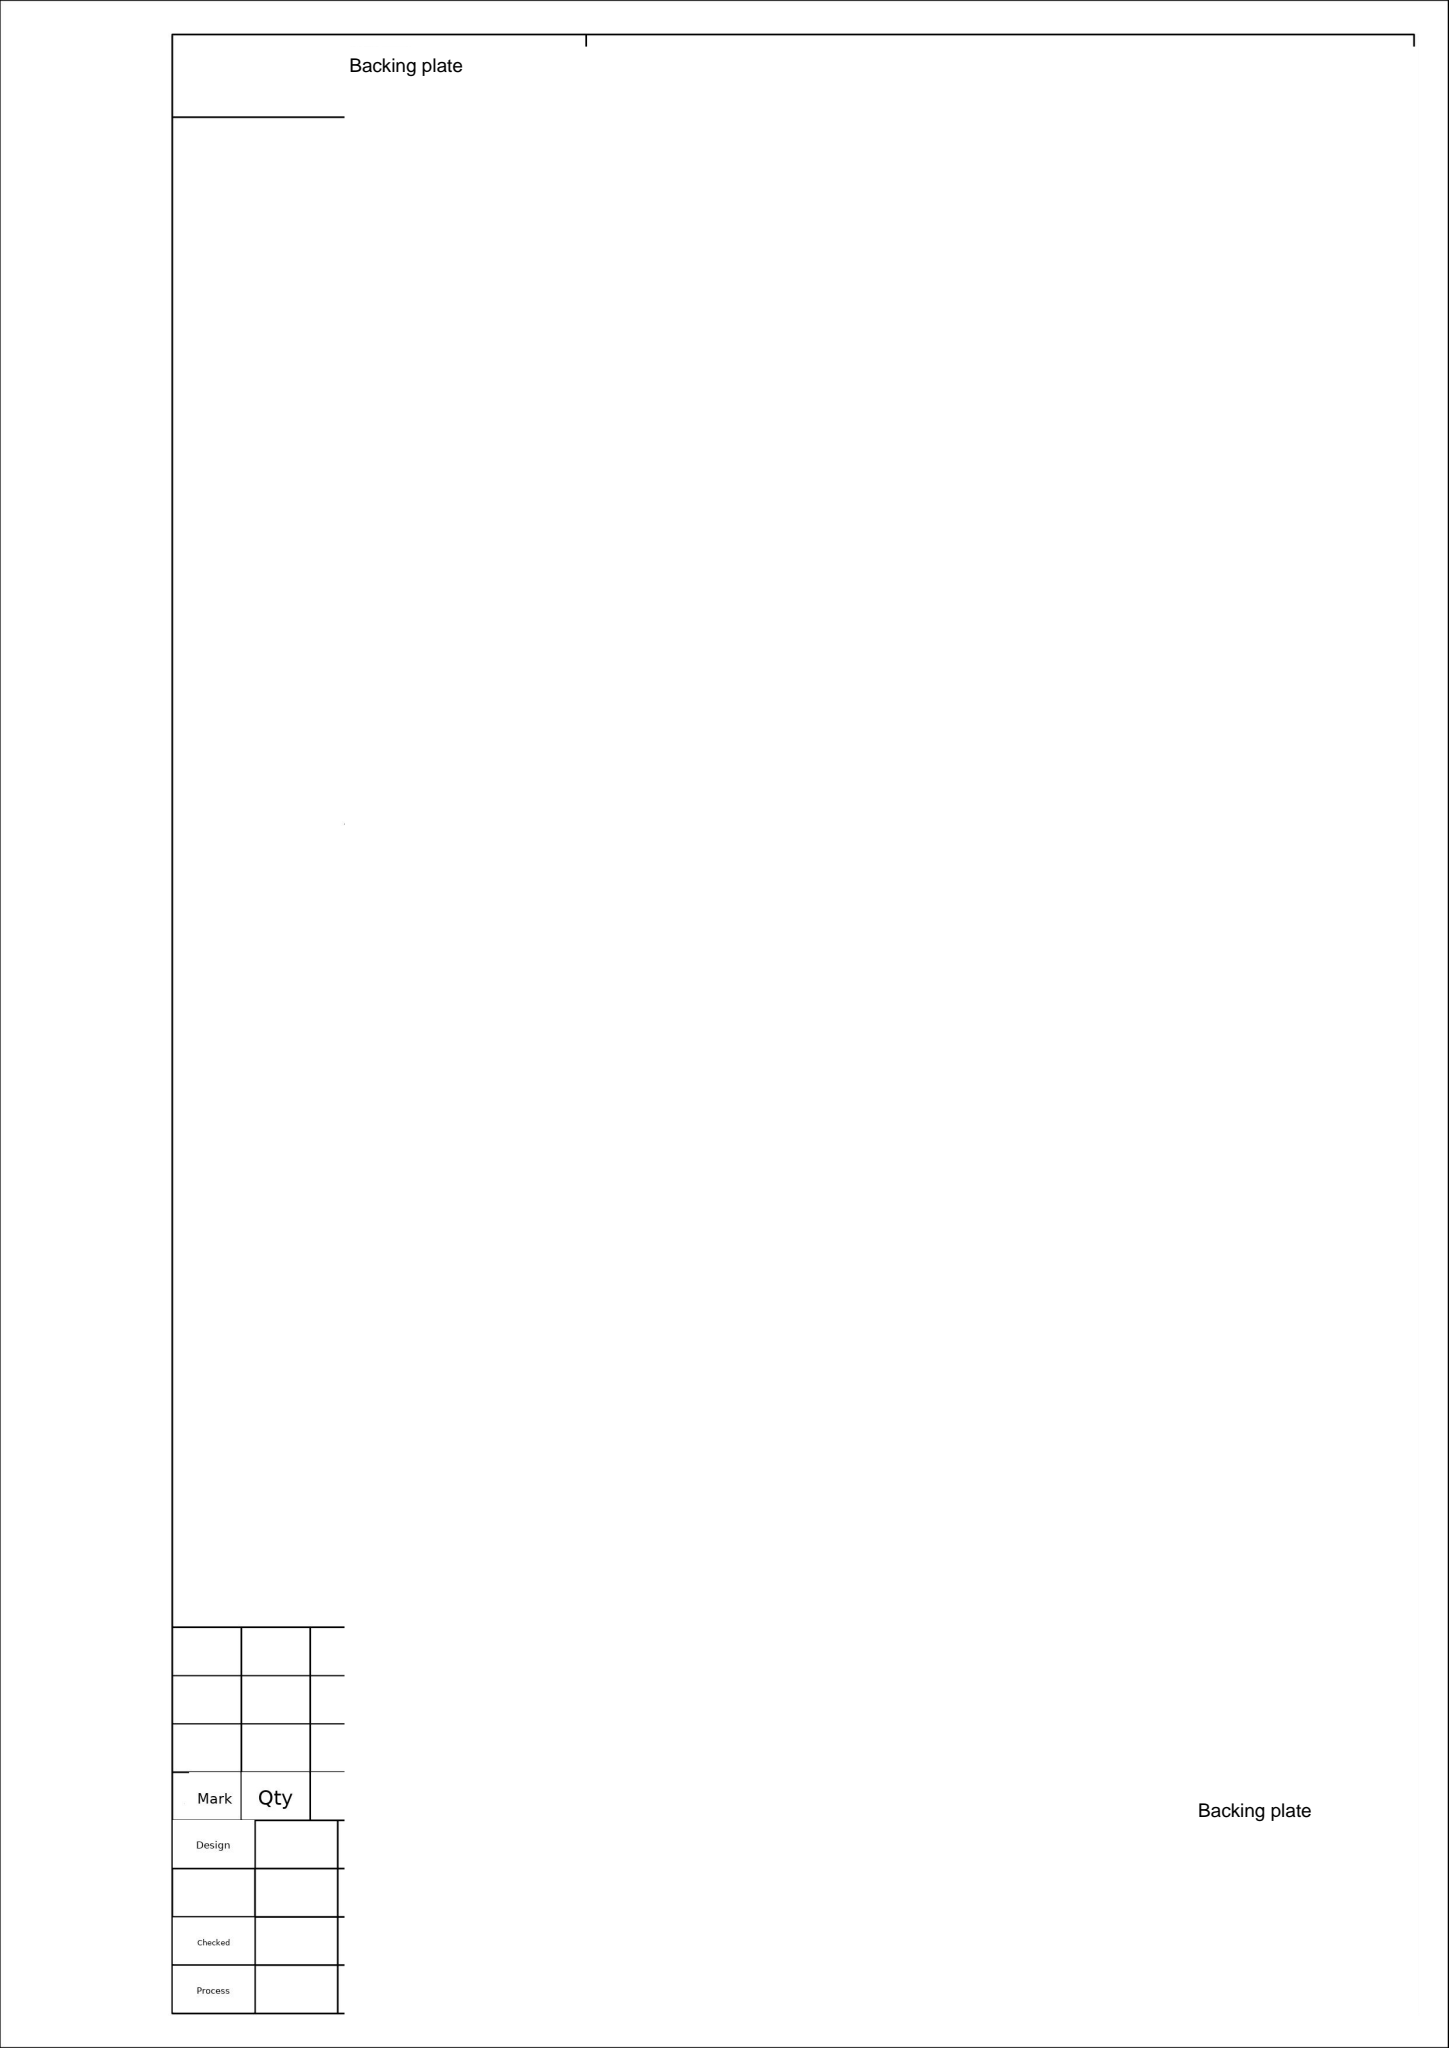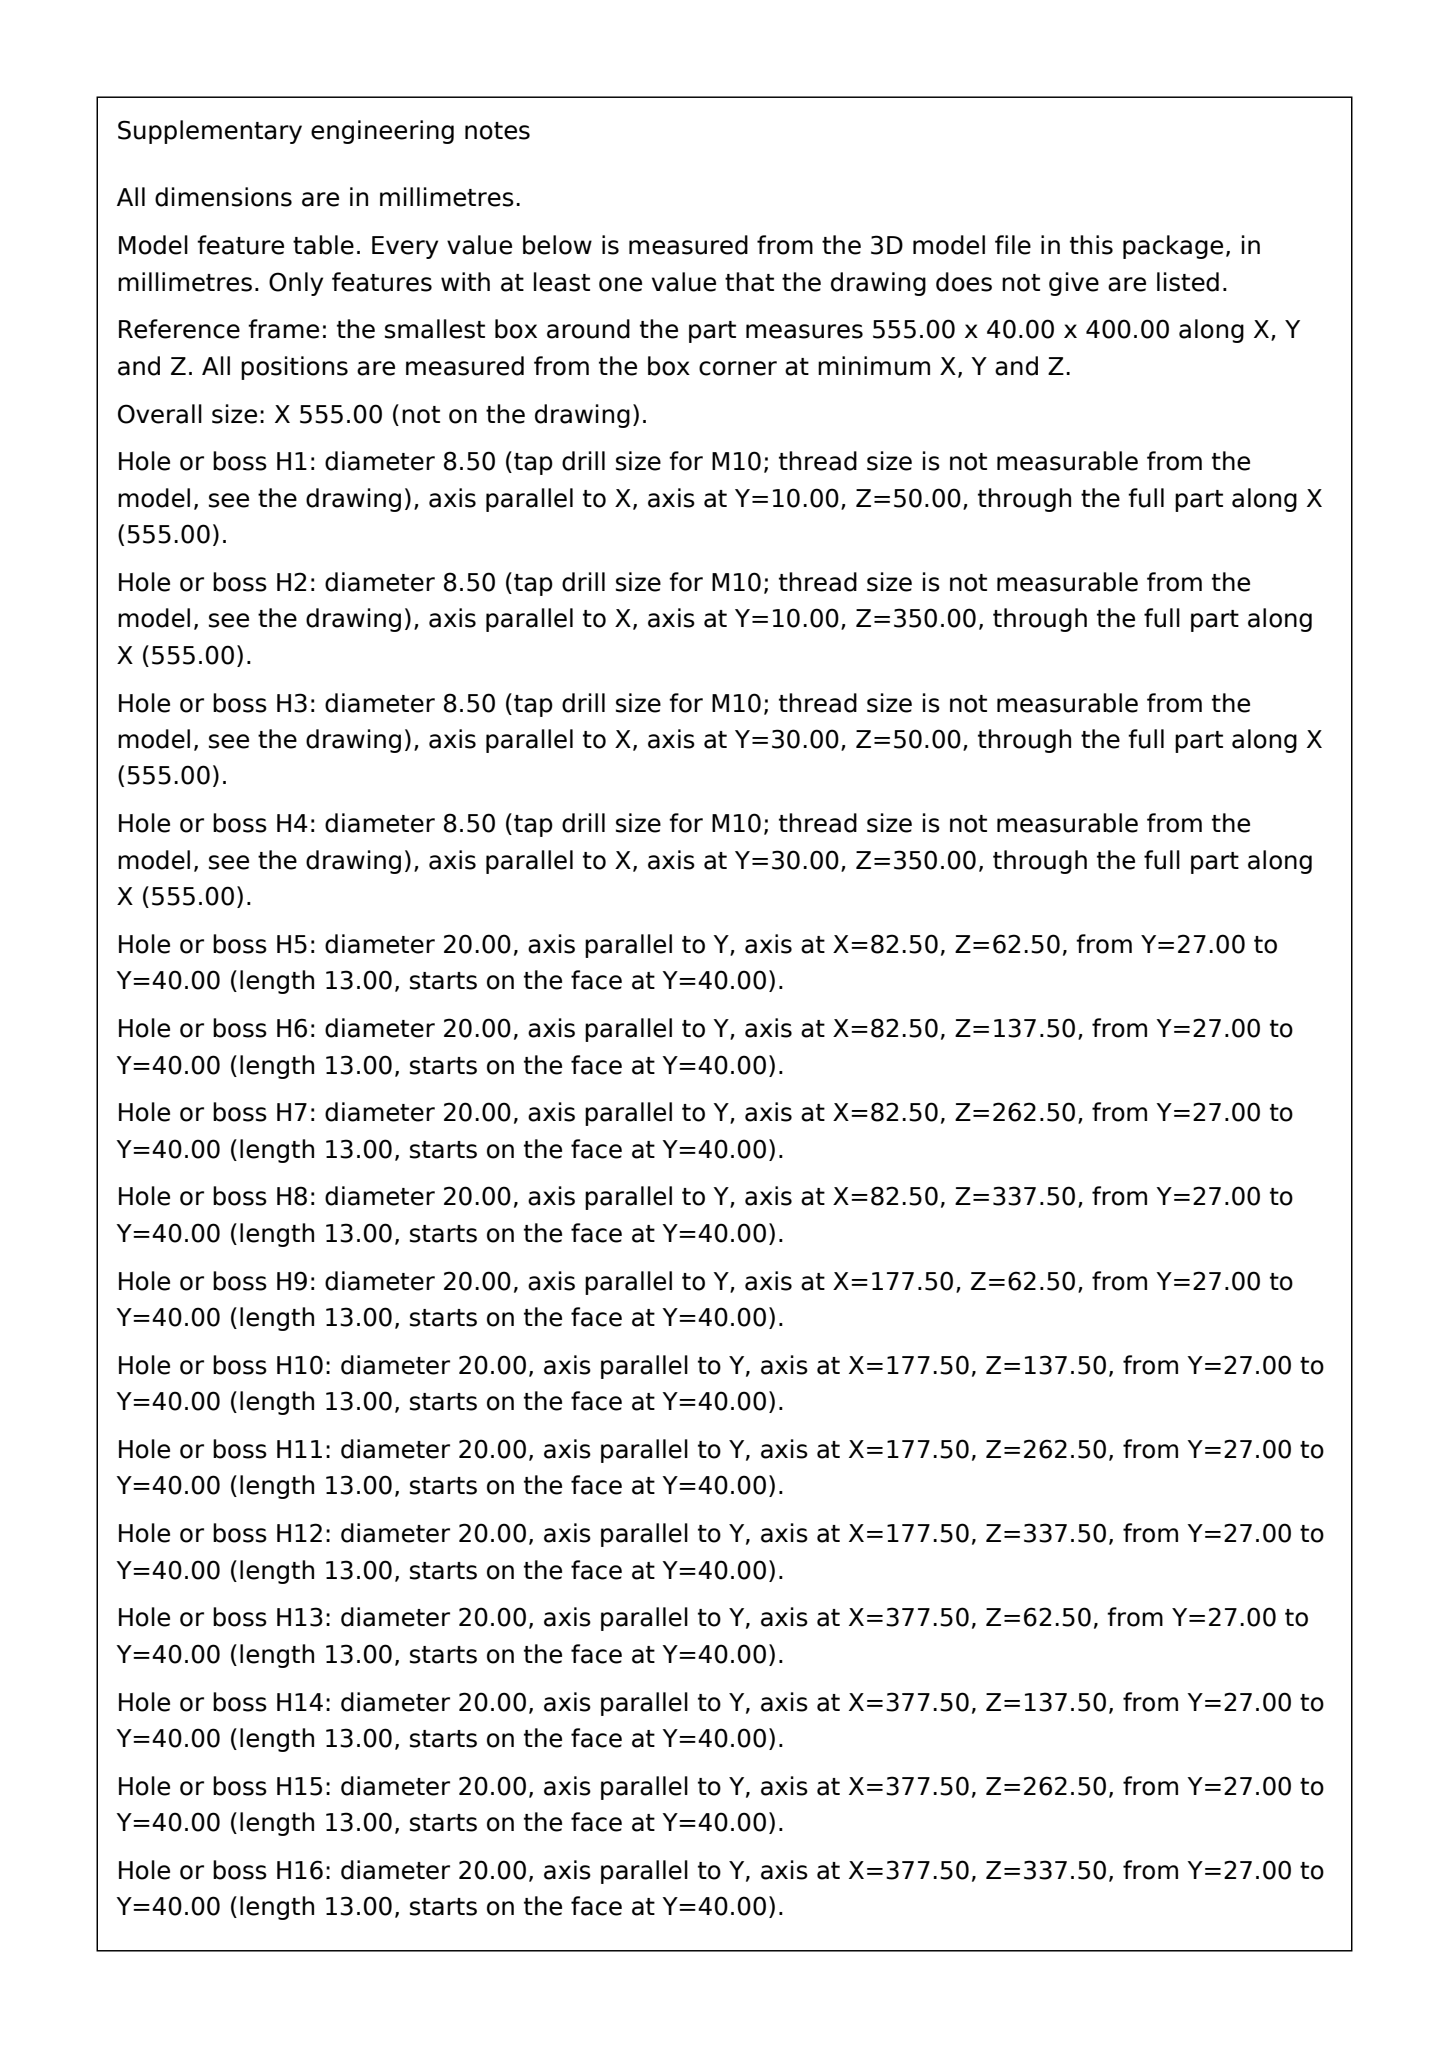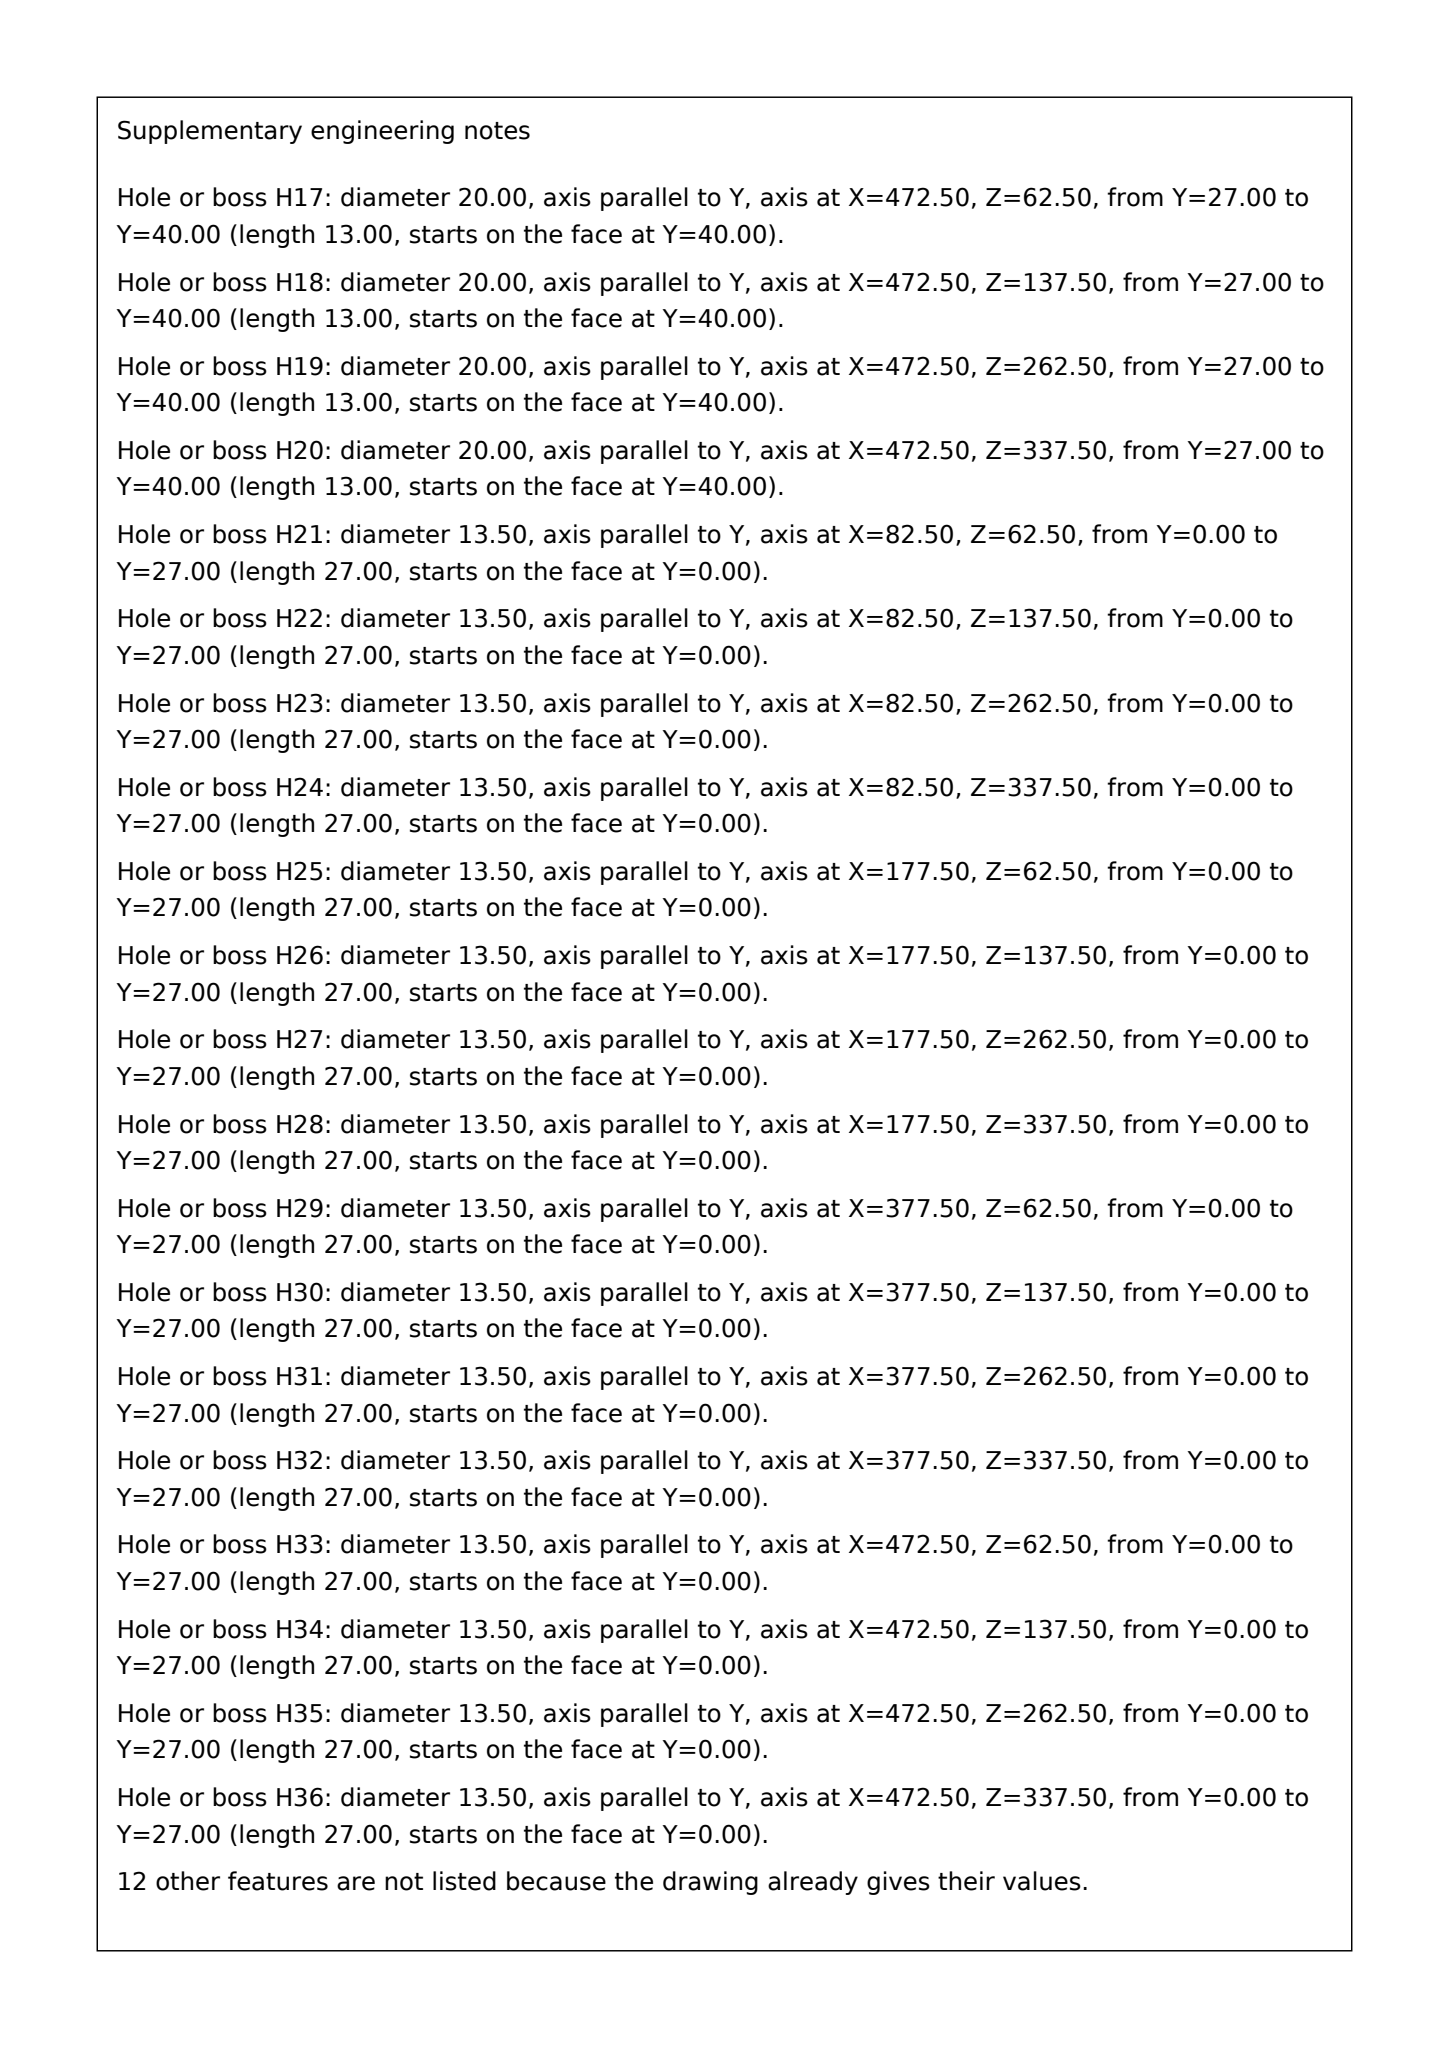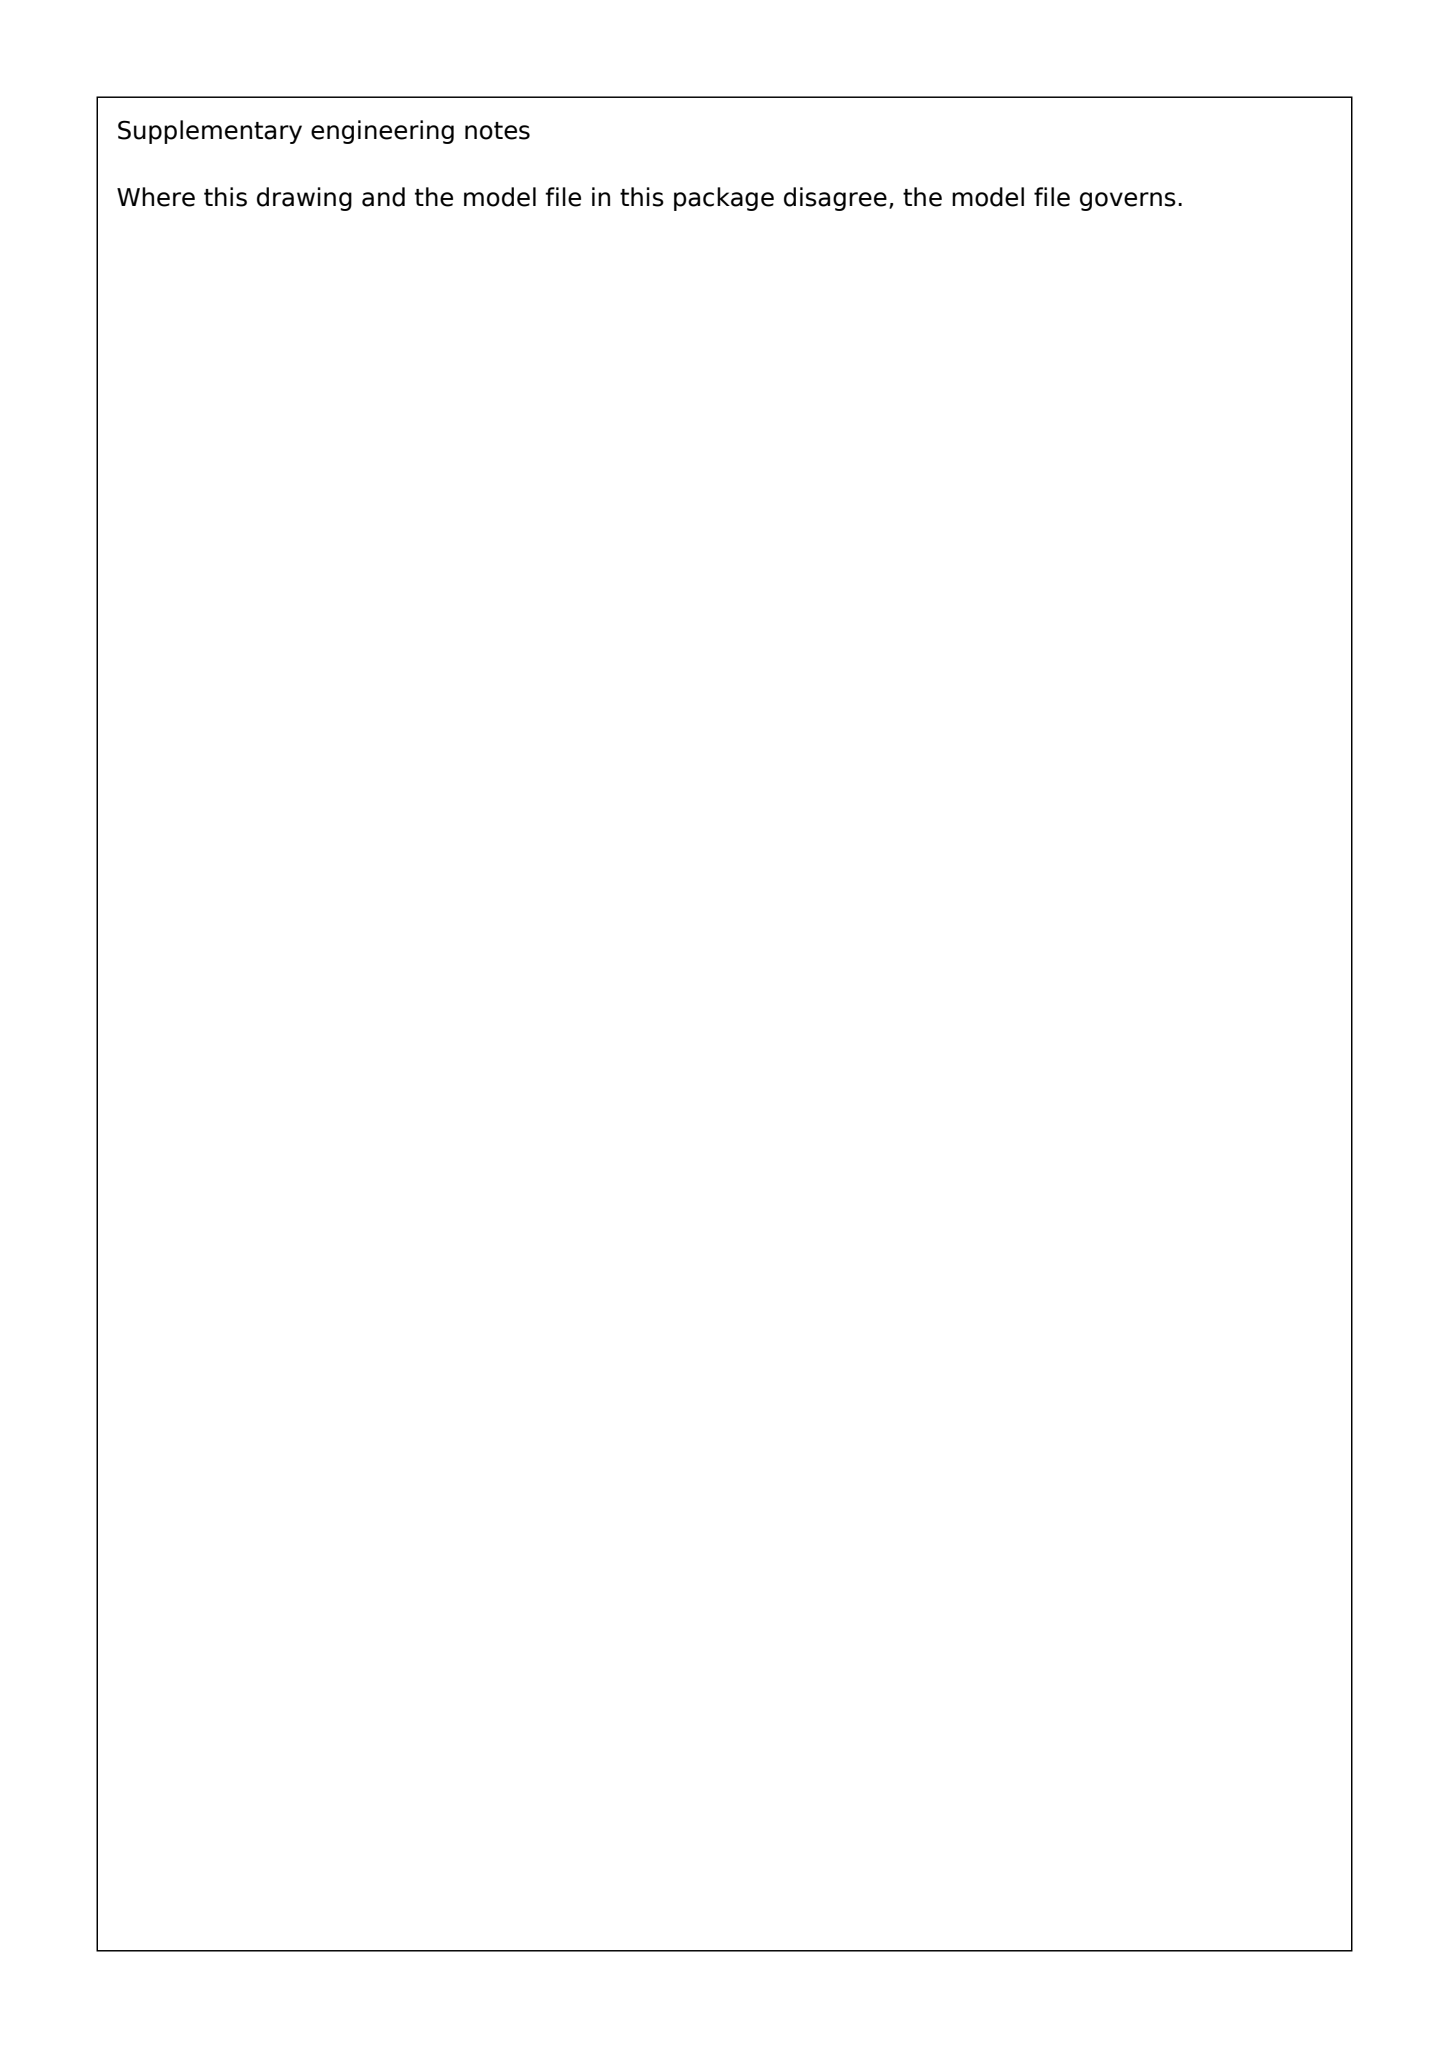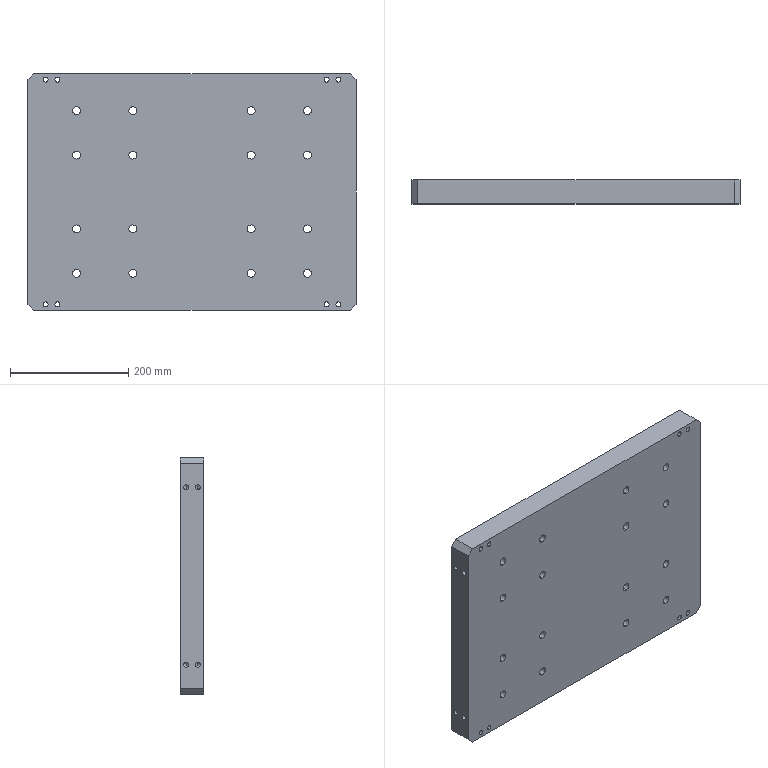Part | SolidWorks | mm | 1 solid | 138 faces | box 555 x 40 x 400 mm | volume 8713790 mm3 | cylinder 96 | plane 26 | cone 16 | commonest cylinder face diameters 8.5 x32 13.5 x32 20 x32
build123d program:
from build123d import *

# Parameters (mm, degrees)
BOSS_EXTRUDE1_DEPTH         = 40
SKETCH3_R                   = 10
CUT_EXTRUDE1_DEPTH          = 13
SKETCH4_R                   = 6.75
CUT_EXTRUDE2_DEPTH          = 345.393
M10_TAPPED_HOLE1_AT_2_COUNT = 2
M10_TAPPED_HOLE1_AT_2_PITCH = 20
CUT_EXTRUDE3_START          = -20
SKETCH8_R                   = 4.25
CUT_EXTRUDE3_DEPTH          = 24.5
MIRROR4_COPY_2_SKETCH_R     = 10
MIRROR4_COPY_2_DEPTH        = 13
MIRROR4_COPY_3_SKETCH_R     = 6.75
MIRROR4_COPY_3_DEPTH        = 345.393
MIRROR4_START               = -20
MIRROR4_COPY_5_SKETCH_R     = 4.25
MIRROR4_COPY_5_DEPTH        = 24.5
M10_TAPPED_HOLE2_AT_2_COUNT = 2
M10_TAPPED_HOLE2_AT_2_PITCH = 20


with BuildPart() as part:
    # Sketch2 → Boss-Extrude1 (new body)
    with BuildSketch(Plane(origin=(0, 0, 0), x_dir=(1, 0, 0), z_dir=(0, 1, 0))):
        Polygon((277.5, -190), (267.5, -200), (-267.5, -200), (-277.5, -190), (-277.5, 190), (-267.5, 200), (267.5, 200), (277.5, 190), align=None)
    extrude(amount=-BOSS_EXTRUDE1_DEPTH)

    # Sketch3 → Cut-Extrude1 (cut)
    with BuildSketch(Plane(origin=(0, 0, 0), x_dir=(1, 0, 0), z_dir=(0, 1, 0))):
        with Locations(Location((-100, -62.5, 0), (0, 0, 270))):
            Circle(SKETCH3_R)
        with Locations(Location((-195, -62.5, 0), (0, 0, 270))):
            Circle(SKETCH3_R)
        with Locations(Location((-195, -137.5, 0), (0, 0, 270))):
            Circle(SKETCH3_R)
        with Locations(Location((-100, -137.5, 0), (0, 0, 270))):
            Circle(SKETCH3_R)
    cut_extrude1 = extrude(amount=-CUT_EXTRUDE1_DEPTH, mode=Mode.SUBTRACT)

    # Sketch4 → Cut-Extrude2 (cut, through all)
    with BuildSketch(Plane(origin=(0, 0, 0), x_dir=(1, 0, 0), z_dir=(0, 1, 0))):
        with Locations(Location((-100, -62.5, 0), (0, 0, 270))):
            Circle(SKETCH4_R)
        with Locations(Location((-195, -62.5, 0), (0, 0, 270))):
            Circle(SKETCH4_R)
        with Locations(Location((-100, -137.5, 0), (0, 0, 270))):
            Circle(SKETCH4_R)
        with Locations(Location((-195, -137.5, 0), (0, 0, 270))):
            Circle(SKETCH4_R)
    cut_extrude2 = extrude(amount=-CUT_EXTRUDE2_DEPTH, mode=Mode.SUBTRACT)

    # Sketch5 → M10 Tapped Hole1 (revolve, cut)
    with BuildSketch(Plane(origin=(-247.5, 0, 190), x_dir=(0, 0, 1), z_dir=(1, 0, 0))):
        Polygon((0, 0), (0, 30.054), (4.25, 27.5), (4.25, 0), align=None)
    m10_tapped_hole1 = revolve(axis=Axis((-247.5, 6.35, 190), (0, -1, 0)), mode=Mode.SUBTRACT)

    # M10 Tapped Hole1 at 2: M10 Tapped Hole1 ×2
    with Locations(*[(i * M10_TAPPED_HOLE1_AT_2_PITCH, 0, 0) for i in range(1, M10_TAPPED_HOLE1_AT_2_COUNT)]):
        add(m10_tapped_hole1, mode=Mode.SUBTRACT)

    # Sketch8 → Cut-Extrude3 (cut)
    with BuildSketch(Plane(origin=(0, 0, 0), x_dir=(1, 0, 0), z_dir=(0, 1, 0)).offset(CUT_EXTRUDE3_START)):
        with Locations(Location((-227.5, -190, 0), (0, 0, 270))):
            Circle(SKETCH8_R)
        with Locations(Location((-247.5, -190, 0), (0, 0, 270))):
            Circle(SKETCH8_R)
    cut_extrude3 = extrude(amount=-CUT_EXTRUDE3_DEPTH, mode=Mode.SUBTRACT)

    # Mirror1: Cut-Extrude1, Cut-Extrude2, M10 Tapped Hole1, Cut-Extrude3 across plane
    add(cut_extrude1.mirror(Plane.XY), mode=Mode.SUBTRACT)
    add(cut_extrude2.mirror(Plane.XY), mode=Mode.SUBTRACT)
    add(m10_tapped_hole1.mirror(Plane.XY), mode=Mode.SUBTRACT)
    add(cut_extrude3.mirror(Plane.XY), mode=Mode.SUBTRACT)

    # Mirror1 copy 1 sketch → Mirror1 copy 1 (revolve, cut)
    with BuildSketch(Plane(origin=(-227.5, 0, -190), x_dir=(0, 0, -1), z_dir=(1, 0, 0))):
        Polygon((0, 0), (0, -30.054), (4.25, -27.5), (4.25, 0), align=None)
    revolve(axis=Axis((-227.5, 6.35, -190), (0, 1, 0)), mode=Mode.SUBTRACT)

    # Mirror4: Cut-Extrude1, Cut-Extrude2, M10 Tapped Hole1, Cut-Extrude3 across plane
    add(cut_extrude1.mirror(Plane(origin=(0, 0, 0), x_dir=(0, 0, 1), z_dir=(1, 0, 0))), mode=Mode.SUBTRACT)
    add(cut_extrude2.mirror(Plane(origin=(0, 0, 0), x_dir=(0, 0, 1), z_dir=(1, 0, 0))), mode=Mode.SUBTRACT)
    add(m10_tapped_hole1.mirror(Plane(origin=(0, 0, 0), x_dir=(0, 0, 1), z_dir=(1, 0, 0))), mode=Mode.SUBTRACT)
    add(cut_extrude3.mirror(Plane(origin=(0, 0, 0), x_dir=(0, 0, 1), z_dir=(1, 0, 0))), mode=Mode.SUBTRACT)

    # Mirror4 copy 1 sketch → Mirror4 copy 1 (revolve, cut)
    with BuildSketch(Plane(origin=(227.5, 0, 190), x_dir=(0, 0, 1), z_dir=(-1, 0, 0))):
        Polygon((0, 0), (0, -30.054), (4.25, -27.5), (4.25, 0), align=None)
    revolve(axis=Axis((227.5, 6.35, 190), (0, 1, 0)), mode=Mode.SUBTRACT)

    # Mirror4 copy 2 sketch → Mirror4 copy 2 (cut)
    with BuildSketch(Plane(origin=(0, 0, 0), x_dir=(-1, 0, 0), z_dir=(0, 1, 0))):
        with Locations(Location((-100, -62.5, 0), (0, 0, 270))):
            Circle(MIRROR4_COPY_2_SKETCH_R)
        with Locations(Location((-195, -62.5, 0), (0, 0, 270))):
            Circle(MIRROR4_COPY_2_SKETCH_R)
        with Locations(Location((-195, -137.5, 0), (0, 0, 270))):
            Circle(MIRROR4_COPY_2_SKETCH_R)
        with Locations(Location((-100, -137.5, 0), (0, 0, 270))):
            Circle(MIRROR4_COPY_2_SKETCH_R)
    extrude(amount=-MIRROR4_COPY_2_DEPTH, mode=Mode.SUBTRACT)

    # Mirror4 copy 3 sketch → Mirror4 copy 3 (cut, through all)
    with BuildSketch(Plane(origin=(0, 0, 0), x_dir=(-1, 0, 0), z_dir=(0, 1, 0))):
        with Locations(Location((-100, -62.5, 0), (0, 0, 270))):
            Circle(MIRROR4_COPY_3_SKETCH_R)
        with Locations(Location((-195, -62.5, 0), (0, 0, 270))):
            Circle(MIRROR4_COPY_3_SKETCH_R)
        with Locations(Location((-100, -137.5, 0), (0, 0, 270))):
            Circle(MIRROR4_COPY_3_SKETCH_R)
        with Locations(Location((-195, -137.5, 0), (0, 0, 270))):
            Circle(MIRROR4_COPY_3_SKETCH_R)
    extrude(amount=-MIRROR4_COPY_3_DEPTH, mode=Mode.SUBTRACT)

    # Mirror4 copy 4 sketch → Mirror4 copy 4 (revolve, cut)
    with BuildSketch(Plane(origin=(247.5, 0, -190), x_dir=(0, 0, -1), z_dir=(-1, 0, 0))):
        Polygon((0, 0), (0, 30.054), (4.25, 27.5), (4.25, 0), align=None)
    revolve(axis=Axis((247.5, 6.35, -190), (0, -1, 0)), mode=Mode.SUBTRACT)

    # Mirror4 copy 5 sketch → Mirror4 copy 5 (cut)
    with BuildSketch(Plane(origin=(0, 0, 0), x_dir=(-1, 0, 0), z_dir=(0, 1, 0)).offset(MIRROR4_START)):
        with Locations(Location((-227.5, -190, 0), (0, 0, 270))):
            Circle(MIRROR4_COPY_5_SKETCH_R)
        with Locations(Location((-247.5, -190, 0), (0, 0, 270))):
            Circle(MIRROR4_COPY_5_SKETCH_R)
    extrude(amount=-MIRROR4_COPY_5_DEPTH, mode=Mode.SUBTRACT)

    # Mirror4 copy 6 sketch → Mirror4 copy 6 (revolve, cut)
    with BuildSketch(Plane(origin=(227.5, 0, -190), x_dir=(0, 0, -1), z_dir=(-1, 0, 0))):
        Polygon((0, 0), (0, 30.054), (4.25, 27.5), (4.25, 0), align=None)
    revolve(axis=Axis((227.5, 6.35, -190), (0, -1, 0)), mode=Mode.SUBTRACT)

    # Sketch7 → M10 Tapped Hole2 (revolve, cut)
    with BuildSketch(Plane(origin=(277.5, -10, 150), x_dir=(0, 0, -1), z_dir=(0, 1, 0))):
        Polygon((0, 0), (0, 30.054), (4.25, 27.5), (4.25, 0), align=None)
    m10_tapped_hole2 = revolve(axis=Axis((283.85, -10, 150), (-1, 0, 0)), mode=Mode.SUBTRACT)

    # M10 Tapped Hole2 at 2: M10 Tapped Hole2 ×2
    with Locations(*[(0, -i * M10_TAPPED_HOLE2_AT_2_PITCH, 0) for i in range(1, M10_TAPPED_HOLE2_AT_2_COUNT)]):
        add(m10_tapped_hole2, mode=Mode.SUBTRACT)

    # Mirror2: M10 Tapped Hole2 across plane
    add(m10_tapped_hole2.mirror(Plane.XY), mode=Mode.SUBTRACT)

    # Mirror2 copy 1 sketch → Mirror2 copy 1 (revolve, cut)
    with BuildSketch(Plane(origin=(277.5, -30, -150), x_dir=(0, 0, 1), z_dir=(0, 1, 0))):
        Polygon((0, 0), (0, -30.054), (4.25, -27.5), (4.25, 0), align=None)
    revolve(axis=Axis((283.85, -30, -150), (1, 0, 0)), mode=Mode.SUBTRACT)

    # Mirror3: M10 Tapped Hole2 across plane
    add(m10_tapped_hole2.mirror(Plane(origin=(0, 0, 0), x_dir=(0, 0, 1), z_dir=(1, 0, 0))), mode=Mode.SUBTRACT)

    # Mirror3 copy 1 sketch → Mirror3 copy 1 (revolve, cut)
    with BuildSketch(Plane(origin=(-277.5, -30, 150), x_dir=(0, 0, -1), z_dir=(0, 1, 0))):
        Polygon((0, 0), (0, -30.054), (4.25, -27.5), (4.25, 0), align=None)
    revolve(axis=Axis((-283.85, -30, 150), (-1, 0, 0)), mode=Mode.SUBTRACT)

    # Mirror3 copy 2 sketch → Mirror3 copy 2 (revolve, cut)
    with BuildSketch(Plane(origin=(-277.5, -10, -150), x_dir=(0, 0, 1), z_dir=(0, 1, 0))):
        Polygon((0, 0), (0, 30.054), (4.25, 27.5), (4.25, 0), align=None)
    revolve(axis=Axis((-283.85, -10, -150), (1, 0, 0)), mode=Mode.SUBTRACT)

    # Mirror3 copy 3 sketch → Mirror3 copy 3 (revolve, cut)
    with BuildSketch(Plane(origin=(-277.5, -30, -150), x_dir=(0, 0, 1), z_dir=(0, 1, 0))):
        Polygon((0, 0), (0, 30.054), (4.25, 27.5), (4.25, 0), align=None)
    revolve(axis=Axis((-283.85, -30, -150), (1, 0, 0)), mode=Mode.SUBTRACT)


solid = part.part